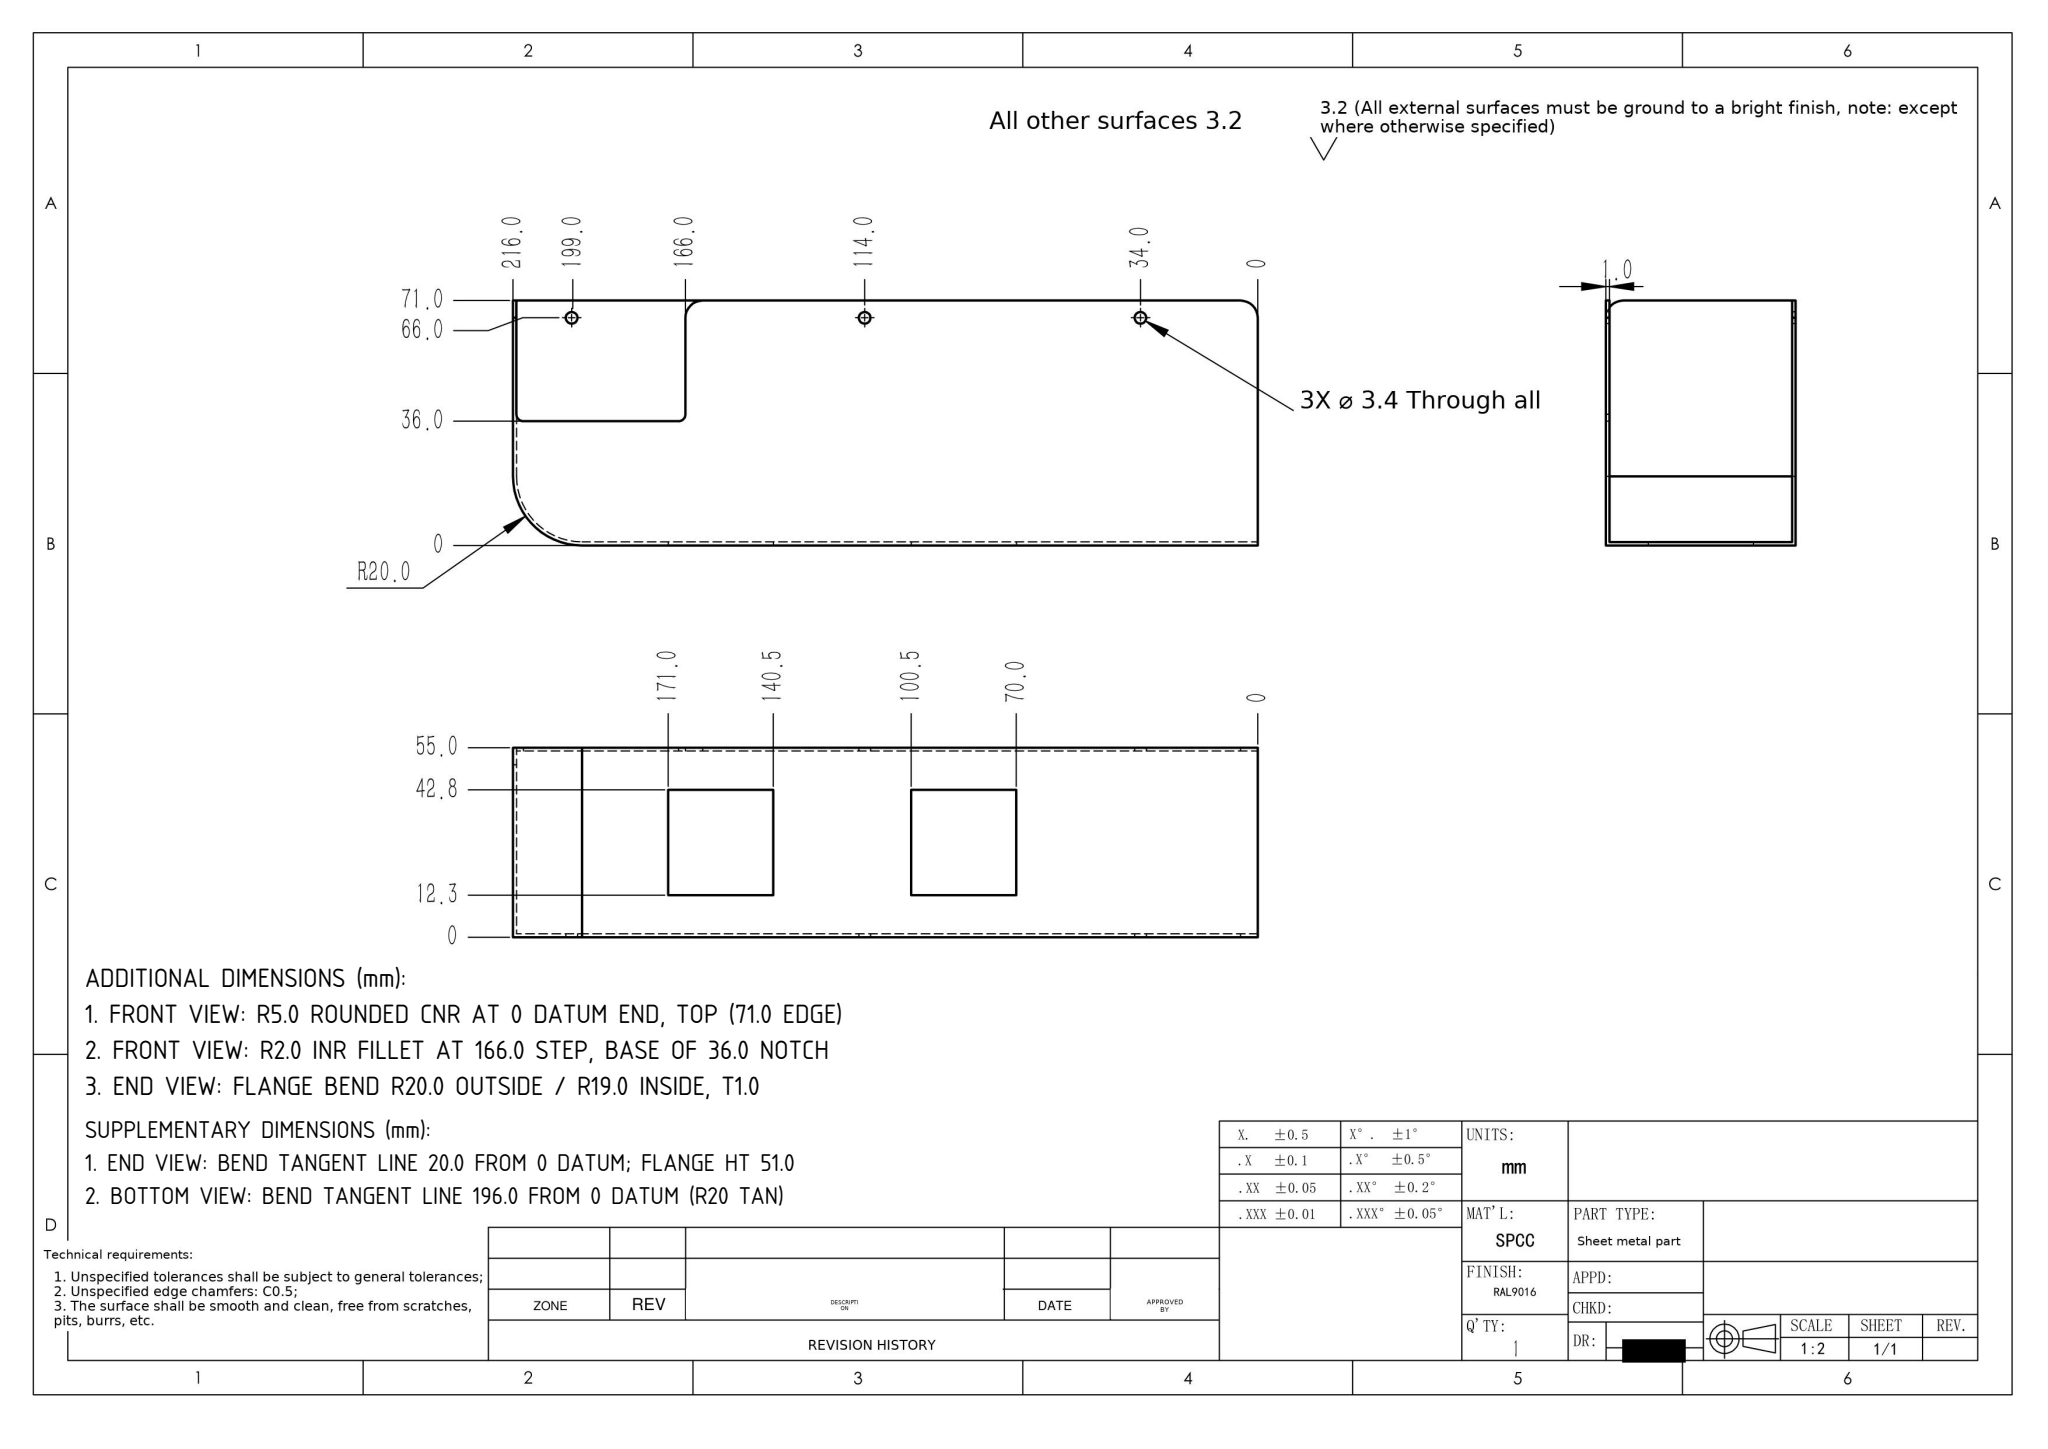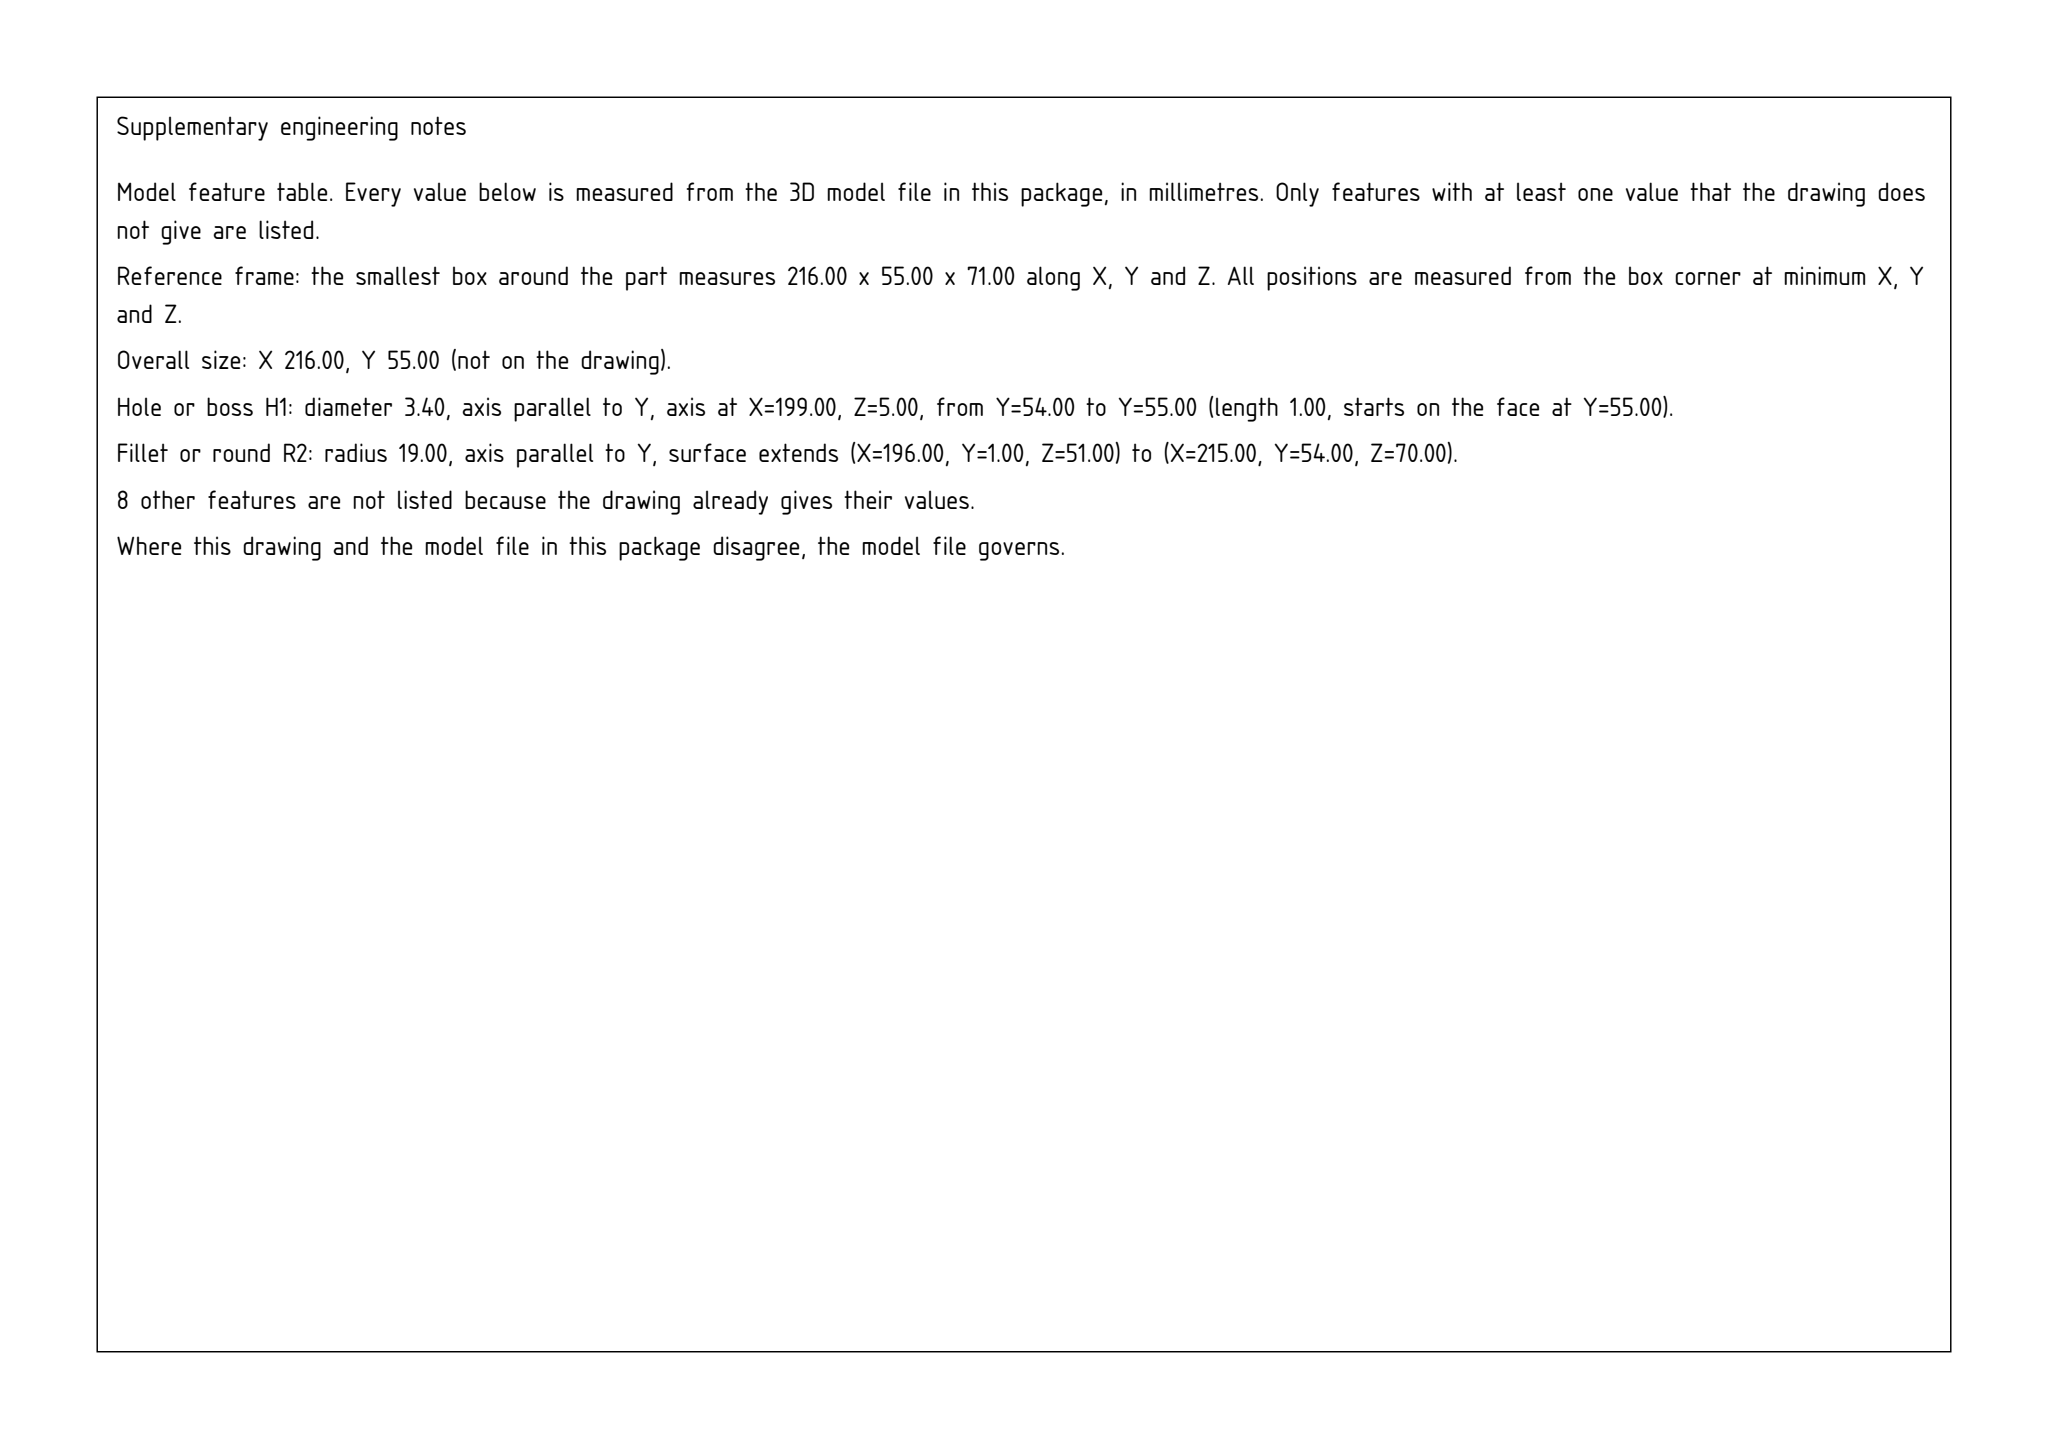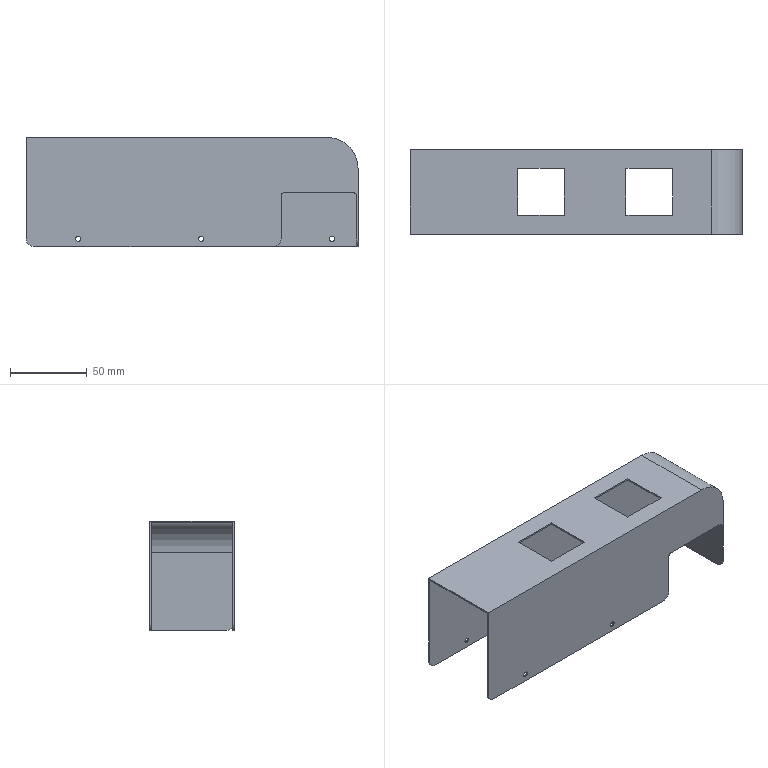Part | SolidWorks | mm | 1 solid | 39 faces | box 216 x 55 x 71 mm | volume 41574 mm3 | plane 21 | cylinder 18 | commonest cylinder face diameters 3.4 x10 10 x4 4 x2 40 x1 38 x1
build123d program:
from build123d import *

# Parameters (mm, degrees)
SKETCH1_W            = 216
SKETCH1_H            = 55
BOSS_EXTRUDE1_DEPTH  = 72
FILLET1_R            = 20
SHELL1_T             = -1
SKETCH2_W            = 216
SKETCH2_H            = 55
CUT_EXTRUDE1_DEPTH   = 1
SKETCH3_W            = 30.5
SKETCH3_H            = 30.5
CUT_EXTRUDE2_DEPTH   = 10
CUT_EXTRUDE3_DEPTH   = 10
M3_CLEARANCE_HOLE1_D = 3.4
FILLET2_R            = 5


with BuildPart() as part:
    # Sketch1 → Boss-Extrude1 (new body)
    with BuildSketch(Plane.XY):
        Rectangle(SKETCH1_W, SKETCH1_H)
    extrude(amount=BOSS_EXTRUDE1_DEPTH)

    # Fillet1
    fillet1_edges = [part.edges().sort_by_distance(p)[0] for p in [
        (108, 0, 72),
    ]]
    fillet(fillet1_edges, radius=FILLET1_R)

    # Shell1
    shell1_openings = [part.faces().sort_by_distance(p)[0] for p in [
        (-108, 0, 36),
    ]]
    offset(amount=SHELL1_T, openings=shell1_openings, kind=Kind.INTERSECTION)

    # Sketch2 → Cut-Extrude1 (cut)
    with BuildSketch(Plane(origin=(0, 0, 0), x_dir=(-1, 0, 0), z_dir=(0, 0, -1))):
        Rectangle(SKETCH2_W, SKETCH2_H)
    extrude(amount=-CUT_EXTRUDE1_DEPTH, mode=Mode.SUBTRACT)

    # Sketch3 → Cut-Extrude2 (cut)
    with BuildSketch(Plane.XY.offset(72)):
        with Locations((47.75, 0)):
            Rectangle(SKETCH3_W, SKETCH3_H)
        with Locations((-22.75, 0)):
            Rectangle(SKETCH3_W, SKETCH3_H)
    extrude(amount=-CUT_EXTRUDE2_DEPTH, mode=Mode.SUBTRACT)

    # Sketch4 → Cut-Extrude3 (cut)
    with BuildSketch(Plane.XZ.offset(27.5)):
        with BuildLine():
            Line((58, 1), (107, 1))
            Line((107, 1), (107, 34))
            ThreePointArc((107, 34), (106.414, 35.414), (105, 36))
            Line((105, 36), (60, 36))
            ThreePointArc((60, 36), (58.586, 35.414), (58, 34))
            Line((58, 34), (58, 1))
        make_face()
    extrude(amount=-CUT_EXTRUDE3_DEPTH, mode=Mode.SUBTRACT)

    # M3 Clearance Hole1 (through all)
    with Locations(Plane(origin=(0, 27.5, 0), x_dir=(1, 0, 0), z_dir=(0, 1, 0))):
        with Locations((91, -6), (6, -6), (-74, -6)):
            Hole(M3_CLEARANCE_HOLE1_D / 2)

    # Fillet2
    fillet2_edges = [part.edges().sort_by_distance(p)[0] for p in [
        (58, -27, 1),
        (107.5, -27.5, 1),
        (-108, -27, 1),
        (-108, 27, 1),
    ]]
    fillet(fillet2_edges, radius=FILLET2_R)


solid = part.part